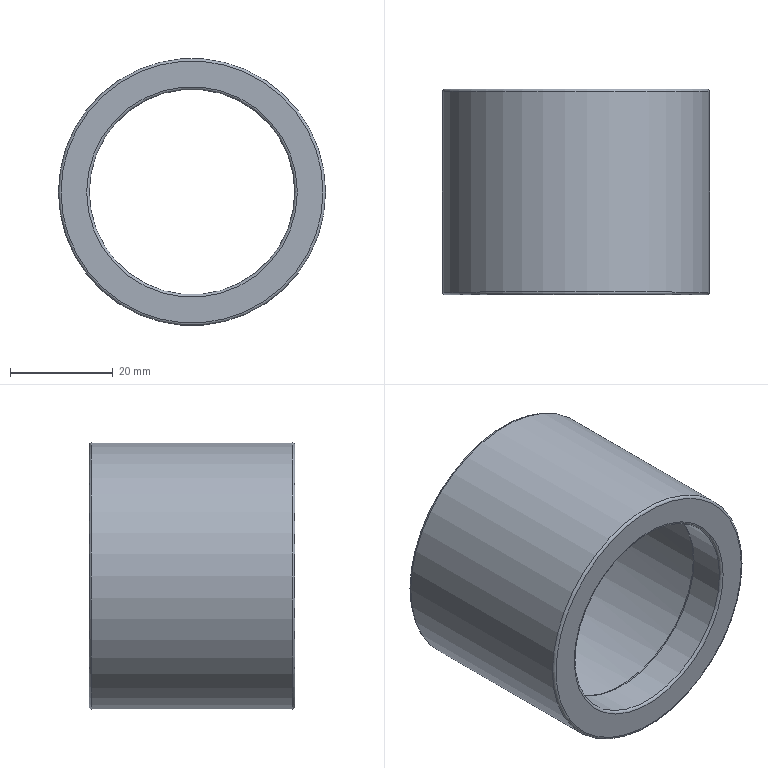Component | NX | 10_THIN_SLEEVE | 1 solid | 16 faces | box 52 x 40 x 52 mm | volume 21385 mm3 | torus 8 | plane 4 | cylinder 4 | commonest cylinder face diameters 40 x2 52 x1 48 x1
STEP:
#1=CARTESIAN_POINT('',(0.,0.,0.));
#2=DIRECTION('',(0.,0.,1.));
#3=DIRECTION('',(1.,0.,0.));
#4=AXIS2_PLACEMENT_3D('',#1,#2,#3);
#5=CARTESIAN_POINT('',(-38.584,152.794,-238.219));
#6=VERTEX_POINT('',#5);
#7=CARTESIAN_POINT('',(-59.084,152.794,-238.219));
#8=DIRECTION('',(0.,-1.,0.));
#9=DIRECTION('',(1.,0.,0.));
#10=AXIS2_PLACEMENT_3D('',#7,#8,#9);
#11=CIRCLE('',#10,20.5);
#12=CARTESIAN_POINT('',(-59.084,152.794,-238.219));
#13=DIRECTION('',(0.,1.,0.));
#14=DIRECTION('',(1.,0.,0.));
#15=AXIS2_PLACEMENT_3D('',#12,#13,#14);
#16=PLANE('',#15);
#17=CARTESIAN_POINT('',(20.5,0.));
#18=CARTESIAN_POINT('',(20.5,-35.507));
#19=CARTESIAN_POINT('',(-10.25,-17.754));
#20=CARTESIAN_POINT('',(-41.,-0.));
#21=CARTESIAN_POINT('',(-10.25,17.754));
#22=CARTESIAN_POINT('',(20.5,35.507));
#23=CARTESIAN_POINT('',(20.5,0.));
#24=(BOUNDED_CURVE()B_SPLINE_CURVE(2,(#17,#18,#19,#20,#21,#22,#23),.UNSPECIFIED.,.T.,.F.)B_SPLINE_CURVE_WITH_KNOTS((1,2,2,2,2,1),(-2.094,0.,2.094,4.189,6.283,8.378),.UNSPECIFIED.)CURVE()GEOMETRIC_REPRESENTATION_ITEM()RATIONAL_B_SPLINE_CURVE((1.,0.5,1.,0.5,1.,0.5,1.))REPRESENTATION_ITEM(''));
#25=(GEOMETRIC_REPRESENTATION_CONTEXT(2)PARAMETRIC_REPRESENTATION_CONTEXT()REPRESENTATION_CONTEXT('',''));
#26=DEFINITIONAL_REPRESENTATION('',(#24),#25);
#27=PCURVE('',#16,#26);
#28=CARTESIAN_POINT('',(-59.084,152.294,-238.219));
#29=DIRECTION('',(0.,1.,0.));
#30=DIRECTION('',(1.,0.,0.));
#31=AXIS2_PLACEMENT_3D('',#28,#29,#30);
#32=TOROIDAL_SURFACE('',#31,20.5,0.5);
#33=CARTESIAN_POINT('',(6.283,7.854));
#34=DIRECTION('',(-1.,0.));
#35=VECTOR('',#34,1.);
#36=LINE('',#33,#35);
#37=(GEOMETRIC_REPRESENTATION_CONTEXT(2)PARAMETRIC_REPRESENTATION_CONTEXT()REPRESENTATION_CONTEXT('',''));
#38=DEFINITIONAL_REPRESENTATION('',(#36),#37);
#39=PCURVE('',#32,#38);
#40=SURFACE_CURVE('',#11,(#27,#39),.PCURVE_S1.);
#41=EDGE_CURVE('',#6,#6,#40,.T.);
#42=ORIENTED_EDGE('',*,*,#41,.T.);
#43=EDGE_LOOP('',(#42));
#44=FACE_BOUND('',#43,.T.);
#45=CARTESIAN_POINT('',(-33.584,152.794,-238.219));
#46=VERTEX_POINT('',#45);
#47=CARTESIAN_POINT('',(-59.084,152.794,-238.219));
#48=DIRECTION('',(0.,1.,0.));
#49=DIRECTION('',(1.,0.,0.));
#50=AXIS2_PLACEMENT_3D('',#47,#48,#49);
#51=CIRCLE('',#50,25.5);
#52=CARTESIAN_POINT('',(0.,0.));
#53=DIRECTION('',(1.,0.));
#54=AXIS2_PLACEMENT_2D('',#52,#53);
#55=CIRCLE('',#54,25.5);
#56=(GEOMETRIC_REPRESENTATION_CONTEXT(2)PARAMETRIC_REPRESENTATION_CONTEXT()REPRESENTATION_CONTEXT('',''));
#57=DEFINITIONAL_REPRESENTATION('',(#55),#56);
#58=PCURVE('',#16,#57);
#59=CARTESIAN_POINT('',(-59.084,152.294,-238.219));
#60=DIRECTION('',(0.,1.,0.));
#61=DIRECTION('',(1.,0.,0.));
#62=AXIS2_PLACEMENT_3D('',#59,#60,#61);
#63=TOROIDAL_SURFACE('',#62,25.5,0.5);
#64=CARTESIAN_POINT('',(0.,7.854));
#65=DIRECTION('',(1.,0.));
#66=VECTOR('',#65,1.);
#67=LINE('',#64,#66);
#68=(GEOMETRIC_REPRESENTATION_CONTEXT(2)PARAMETRIC_REPRESENTATION_CONTEXT()REPRESENTATION_CONTEXT('',''));
#69=DEFINITIONAL_REPRESENTATION('',(#67),#68);
#70=PCURVE('',#63,#69);
#71=SURFACE_CURVE('',#51,(#58,#70),.PCURVE_S1.);
#72=EDGE_CURVE('',#46,#46,#71,.T.);
#73=ORIENTED_EDGE('',*,*,#72,.T.);
#74=EDGE_LOOP('',(#73));
#75=FACE_BOUND('',#74,.T.);
#76=ADVANCED_FACE('',(#44,#75),#16,.T.);
#77=CARTESIAN_POINT('',(-79.584,112.794,-238.219));
#78=VERTEX_POINT('',#77);
#79=CARTESIAN_POINT('',(-59.084,112.794,-238.219));
#80=DIRECTION('',(0.,1.,0.));
#81=DIRECTION('',(-1.,0.,0.));
#82=AXIS2_PLACEMENT_3D('',#79,#80,#81);
#83=CIRCLE('',#82,20.5);
#84=CARTESIAN_POINT('',(-59.084,112.794,-238.219));
#85=DIRECTION('',(0.,-1.,0.));
#86=DIRECTION('',(-1.,0.,0.));
#87=AXIS2_PLACEMENT_3D('',#84,#85,#86);
#88=PLANE('',#87);
#89=CARTESIAN_POINT('',(20.5,0.));
#90=CARTESIAN_POINT('',(20.5,-35.507));
#91=CARTESIAN_POINT('',(-10.25,-17.754));
#92=CARTESIAN_POINT('',(-41.,-0.));
#93=CARTESIAN_POINT('',(-10.25,17.754));
#94=CARTESIAN_POINT('',(20.5,35.507));
#95=CARTESIAN_POINT('',(20.5,0.));
#96=(BOUNDED_CURVE()B_SPLINE_CURVE(2,(#89,#90,#91,#92,#93,#94,#95),.UNSPECIFIED.,.T.,.F.)B_SPLINE_CURVE_WITH_KNOTS((1,2,2,2,2,1),(-2.094,0.,2.094,4.189,6.283,8.378),.UNSPECIFIED.)CURVE()GEOMETRIC_REPRESENTATION_ITEM()RATIONAL_B_SPLINE_CURVE((1.,0.5,1.,0.5,1.,0.5,1.))REPRESENTATION_ITEM(''));
#97=(GEOMETRIC_REPRESENTATION_CONTEXT(2)PARAMETRIC_REPRESENTATION_CONTEXT()REPRESENTATION_CONTEXT('',''));
#98=DEFINITIONAL_REPRESENTATION('',(#96),#97);
#99=PCURVE('',#88,#98);
#100=CARTESIAN_POINT('',(-59.084,113.294,-238.219));
#101=DIRECTION('',(0.,-1.,0.));
#102=DIRECTION('',(-1.,0.,0.));
#103=AXIS2_PLACEMENT_3D('',#100,#101,#102);
#104=TOROIDAL_SURFACE('',#103,20.5,0.5);
#105=CARTESIAN_POINT('',(6.283,7.854));
#106=DIRECTION('',(-1.,0.));
#107=VECTOR('',#106,1.);
#108=LINE('',#105,#107);
#109=(GEOMETRIC_REPRESENTATION_CONTEXT(2)PARAMETRIC_REPRESENTATION_CONTEXT()REPRESENTATION_CONTEXT('',''));
#110=DEFINITIONAL_REPRESENTATION('',(#108),#109);
#111=PCURVE('',#104,#110);
#112=SURFACE_CURVE('',#83,(#99,#111),.PCURVE_S1.);
#113=EDGE_CURVE('',#78,#78,#112,.T.);
#114=ORIENTED_EDGE('',*,*,#113,.T.);
#115=EDGE_LOOP('',(#114));
#116=FACE_BOUND('',#115,.T.);
#117=CARTESIAN_POINT('',(-84.584,112.794,-238.219));
#118=VERTEX_POINT('',#117);
#119=CARTESIAN_POINT('',(-59.084,112.794,-238.219));
#120=DIRECTION('',(0.,-1.,0.));
#121=DIRECTION('',(-1.,0.,0.));
#122=AXIS2_PLACEMENT_3D('',#119,#120,#121);
#123=CIRCLE('',#122,25.5);
#124=CARTESIAN_POINT('',(0.,0.));
#125=DIRECTION('',(1.,0.));
#126=AXIS2_PLACEMENT_2D('',#124,#125);
#127=CIRCLE('',#126,25.5);
#128=(GEOMETRIC_REPRESENTATION_CONTEXT(2)PARAMETRIC_REPRESENTATION_CONTEXT()REPRESENTATION_CONTEXT('',''));
#129=DEFINITIONAL_REPRESENTATION('',(#127),#128);
#130=PCURVE('',#88,#129);
#131=CARTESIAN_POINT('',(-59.084,113.294,-238.219));
#132=DIRECTION('',(0.,-1.,0.));
#133=DIRECTION('',(-1.,0.,0.));
#134=AXIS2_PLACEMENT_3D('',#131,#132,#133);
#135=TOROIDAL_SURFACE('',#134,25.5,0.5);
#136=CARTESIAN_POINT('',(0.,7.854));
#137=DIRECTION('',(1.,0.));
#138=VECTOR('',#137,1.);
#139=LINE('',#136,#138);
#140=(GEOMETRIC_REPRESENTATION_CONTEXT(2)PARAMETRIC_REPRESENTATION_CONTEXT()REPRESENTATION_CONTEXT('',''));
#141=DEFINITIONAL_REPRESENTATION('',(#139),#140);
#142=PCURVE('',#135,#141);
#143=SURFACE_CURVE('',#123,(#130,#142),.PCURVE_S1.);
#144=EDGE_CURVE('',#118,#118,#143,.T.);
#145=ORIENTED_EDGE('',*,*,#144,.T.);
#146=EDGE_LOOP('',(#145));
#147=FACE_BOUND('',#146,.T.);
#148=ADVANCED_FACE('',(#116,#147),#88,.T.);
#149=CARTESIAN_POINT('',(-85.084,113.294,-238.219));
#150=VERTEX_POINT('',#149);
#151=CARTESIAN_POINT('',(-33.084,113.294,-238.219));
#152=VERTEX_POINT('',#151);
#153=CARTESIAN_POINT('',(-59.084,113.294,-238.219));
#154=DIRECTION('',(0.,1.,0.));
#155=DIRECTION('',(-1.,0.,0.));
#156=AXIS2_PLACEMENT_3D('',#153,#154,#155);
#157=CIRCLE('',#156,26.);
#158=CARTESIAN_POINT('',(-59.084,112.794,-238.219));
#159=DIRECTION('',(0.,1.,0.));
#160=DIRECTION('',(1.,0.,0.));
#161=AXIS2_PLACEMENT_3D('',#158,#159,#160);
#162=CYLINDRICAL_SURFACE('',#161,26.);
#163=CARTESIAN_POINT('',(3.142,0.5));
#164=DIRECTION('',(1.,0.));
#165=VECTOR('',#164,1.);
#166=LINE('',#163,#165);
#167=(GEOMETRIC_REPRESENTATION_CONTEXT(2)PARAMETRIC_REPRESENTATION_CONTEXT()REPRESENTATION_CONTEXT('',''));
#168=DEFINITIONAL_REPRESENTATION('',(#166),#167);
#169=PCURVE('',#162,#168);
#170=CARTESIAN_POINT('',(6.283,6.283));
#171=DIRECTION('',(-1.,0.));
#172=VECTOR('',#171,1.);
#173=LINE('',#170,#172);
#174=(GEOMETRIC_REPRESENTATION_CONTEXT(2)PARAMETRIC_REPRESENTATION_CONTEXT()REPRESENTATION_CONTEXT('',''));
#175=DEFINITIONAL_REPRESENTATION('',(#173),#174);
#176=PCURVE('',#135,#175);
#177=SURFACE_CURVE('',#157,(#169,#176),.PCURVE_S1.);
#178=EDGE_CURVE('',#150,#152,#177,.T.);
#179=ORIENTED_EDGE('',*,*,#178,.T.);
#180=CARTESIAN_POINT('',(-33.084,152.294,-238.219));
#181=VERTEX_POINT('',#180);
#182=CARTESIAN_POINT('',(-33.084,113.294,-238.219));
#183=CARTESIAN_POINT('',(-33.084,152.294,-238.219));
#184=B_SPLINE_CURVE_WITH_KNOTS('',1,(#182,#183),.UNSPECIFIED.,.F.,.F.,(2,2),(0.5,39.5),.PIECEWISE_BEZIER_KNOTS.);
#185=CARTESIAN_POINT('',(6.283,0.));
#186=DIRECTION('',(0.,1.));
#187=VECTOR('',#186,1.);
#188=LINE('',#185,#187);
#189=(GEOMETRIC_REPRESENTATION_CONTEXT(2)PARAMETRIC_REPRESENTATION_CONTEXT()REPRESENTATION_CONTEXT('',''));
#190=DEFINITIONAL_REPRESENTATION('',(#188),#189);
#191=PCURVE('',#162,#190);
#192=CARTESIAN_POINT('',(0.,0.));
#193=DIRECTION('',(0.,1.));
#194=VECTOR('',#193,1.);
#195=LINE('',#192,#194);
#196=(GEOMETRIC_REPRESENTATION_CONTEXT(2)PARAMETRIC_REPRESENTATION_CONTEXT()REPRESENTATION_CONTEXT('',''));
#197=DEFINITIONAL_REPRESENTATION('',(#195),#196);
#198=PCURVE('',#162,#197);
#199=SEAM_CURVE('',#184,(#191,#198),.PCURVE_S1.);
#200=EDGE_CURVE('',#152,#181,#199,.T.);
#201=ORIENTED_EDGE('',*,*,#200,.T.);
#202=CARTESIAN_POINT('',(-59.084,152.294,-238.219));
#203=DIRECTION('',(0.,-1.,0.));
#204=DIRECTION('',(1.,0.,0.));
#205=AXIS2_PLACEMENT_3D('',#202,#203,#204);
#206=CIRCLE('',#205,26.);
#207=CARTESIAN_POINT('',(6.283,39.5));
#208=DIRECTION('',(-1.,0.));
#209=VECTOR('',#208,1.);
#210=LINE('',#207,#209);
#211=(GEOMETRIC_REPRESENTATION_CONTEXT(2)PARAMETRIC_REPRESENTATION_CONTEXT()REPRESENTATION_CONTEXT('',''));
#212=DEFINITIONAL_REPRESENTATION('',(#210),#211);
#213=PCURVE('',#162,#212);
#214=CARTESIAN_POINT('',(6.283,6.283));
#215=DIRECTION('',(-1.,0.));
#216=VECTOR('',#215,1.);
#217=LINE('',#214,#216);
#218=(GEOMETRIC_REPRESENTATION_CONTEXT(2)PARAMETRIC_REPRESENTATION_CONTEXT()REPRESENTATION_CONTEXT('',''));
#219=DEFINITIONAL_REPRESENTATION('',(#217),#218);
#220=PCURVE('',#63,#219);
#221=SURFACE_CURVE('',#206,(#213,#220),.PCURVE_S1.);
#222=EDGE_CURVE('',#181,#181,#221,.T.);
#223=ORIENTED_EDGE('',*,*,#222,.T.);
#224=ORIENTED_EDGE('',*,*,#200,.F.);
#225=CARTESIAN_POINT('',(-59.084,113.294,-238.219));
#226=DIRECTION('',(0.,1.,0.));
#227=DIRECTION('',(-1.,0.,0.));
#228=AXIS2_PLACEMENT_3D('',#225,#226,#227);
#229=CIRCLE('',#228,26.);
#230=CARTESIAN_POINT('',(-3.142,0.5));
#231=DIRECTION('',(1.,0.));
#232=VECTOR('',#231,1.);
#233=LINE('',#230,#232);
#234=(GEOMETRIC_REPRESENTATION_CONTEXT(2)PARAMETRIC_REPRESENTATION_CONTEXT()REPRESENTATION_CONTEXT('',''));
#235=DEFINITIONAL_REPRESENTATION('',(#233),#234);
#236=PCURVE('',#162,#235);
#237=CARTESIAN_POINT('',(6.283,6.283));
#238=DIRECTION('',(-1.,0.));
#239=VECTOR('',#238,1.);
#240=LINE('',#237,#239);
#241=(GEOMETRIC_REPRESENTATION_CONTEXT(2)PARAMETRIC_REPRESENTATION_CONTEXT()REPRESENTATION_CONTEXT('',''));
#242=DEFINITIONAL_REPRESENTATION('',(#240),#241);
#243=PCURVE('',#135,#242);
#244=SURFACE_CURVE('',#229,(#236,#243),.PCURVE_S1.);
#245=EDGE_CURVE('',#152,#150,#244,.T.);
#246=ORIENTED_EDGE('',*,*,#245,.T.);
#247=EDGE_LOOP('',(#179,#201,#223,#224,#246));
#248=FACE_BOUND('',#247,.T.);
#249=ADVANCED_FACE('',(#248),#162,.T.);
#250=CARTESIAN_POINT('',(-79.084,120.294,-238.219));
#251=VERTEX_POINT('',#250);
#252=CARTESIAN_POINT('',(-59.084,120.294,-238.219));
#253=DIRECTION('',(0.,1.,0.));
#254=DIRECTION('',(-1.,0.,0.));
#255=AXIS2_PLACEMENT_3D('',#252,#253,#254);
#256=CIRCLE('',#255,20.);
#257=CARTESIAN_POINT('',(-59.084,112.794,-238.219));
#258=DIRECTION('',(0.,1.,0.));
#259=DIRECTION('',(1.,0.,0.));
#260=AXIS2_PLACEMENT_3D('',#257,#258,#259);
#261=CYLINDRICAL_SURFACE('',#260,20.);
#262=CARTESIAN_POINT('',(3.142,7.5));
#263=DIRECTION('',(1.,0.));
#264=VECTOR('',#263,1.);
#265=LINE('',#262,#264);
#266=(GEOMETRIC_REPRESENTATION_CONTEXT(2)PARAMETRIC_REPRESENTATION_CONTEXT()REPRESENTATION_CONTEXT('',''));
#267=DEFINITIONAL_REPRESENTATION('',(#265),#266);
#268=PCURVE('',#261,#267);
#269=CARTESIAN_POINT('',(-59.084,120.294,-238.219));
#270=DIRECTION('',(0.,-1.,0.));
#271=DIRECTION('',(-1.,0.,0.));
#272=AXIS2_PLACEMENT_3D('',#269,#270,#271);
#273=TOROIDAL_SURFACE('',#272,20.5,0.5);
#274=CARTESIAN_POINT('',(6.283,3.142));
#275=DIRECTION('',(-1.,0.));
#276=VECTOR('',#275,1.);
#277=LINE('',#274,#276);
#278=(GEOMETRIC_REPRESENTATION_CONTEXT(2)PARAMETRIC_REPRESENTATION_CONTEXT()REPRESENTATION_CONTEXT('',''));
#279=DEFINITIONAL_REPRESENTATION('',(#277),#278);
#280=PCURVE('',#273,#279);
#281=SURFACE_CURVE('',#256,(#268,#280),.PCURVE_S1.);
#282=EDGE_CURVE('',#251,#251,#281,.T.);
#283=ORIENTED_EDGE('',*,*,#282,.F.);
#284=CARTESIAN_POINT('',(-79.084,113.294,-238.219));
#285=VERTEX_POINT('',#284);
#286=CARTESIAN_POINT('',(-79.084,113.294,-238.219));
#287=CARTESIAN_POINT('',(-79.084,120.294,-238.219));
#288=B_SPLINE_CURVE_WITH_KNOTS('',1,(#286,#287),.UNSPECIFIED.,.F.,.F.,(2,2),(0.5,7.5),.PIECEWISE_BEZIER_KNOTS.);
#289=CARTESIAN_POINT('',(3.142,0.));
#290=DIRECTION('',(0.,1.));
#291=VECTOR('',#290,1.);
#292=LINE('',#289,#291);
#293=(GEOMETRIC_REPRESENTATION_CONTEXT(2)PARAMETRIC_REPRESENTATION_CONTEXT()REPRESENTATION_CONTEXT('',''));
#294=DEFINITIONAL_REPRESENTATION('',(#292),#293);
#295=PCURVE('',#261,#294);
#296=CARTESIAN_POINT('',(9.425,0.));
#297=DIRECTION('',(0.,1.));
#298=VECTOR('',#297,1.);
#299=LINE('',#296,#298);
#300=(GEOMETRIC_REPRESENTATION_CONTEXT(2)PARAMETRIC_REPRESENTATION_CONTEXT()REPRESENTATION_CONTEXT('',''));
#301=DEFINITIONAL_REPRESENTATION('',(#299),#300);
#302=PCURVE('',#261,#301);
#303=SEAM_CURVE('',#288,(#295,#302),.PCURVE_S1.);
#304=EDGE_CURVE('',#285,#251,#303,.T.);
#305=ORIENTED_EDGE('',*,*,#304,.F.);
#306=CARTESIAN_POINT('',(-59.084,113.294,-238.219));
#307=DIRECTION('',(0.,-1.,0.));
#308=DIRECTION('',(-1.,0.,0.));
#309=AXIS2_PLACEMENT_3D('',#306,#307,#308);
#310=CIRCLE('',#309,20.);
#311=CARTESIAN_POINT('',(9.425,0.5));
#312=DIRECTION('',(-1.,0.));
#313=VECTOR('',#312,1.);
#314=LINE('',#311,#313);
#315=(GEOMETRIC_REPRESENTATION_CONTEXT(2)PARAMETRIC_REPRESENTATION_CONTEXT()REPRESENTATION_CONTEXT('',''));
#316=DEFINITIONAL_REPRESENTATION('',(#314),#315);
#317=PCURVE('',#261,#316);
#318=CARTESIAN_POINT('',(0.,9.425));
#319=DIRECTION('',(1.,0.));
#320=VECTOR('',#319,1.);
#321=LINE('',#318,#320);
#322=(GEOMETRIC_REPRESENTATION_CONTEXT(2)PARAMETRIC_REPRESENTATION_CONTEXT()REPRESENTATION_CONTEXT('',''));
#323=DEFINITIONAL_REPRESENTATION('',(#321),#322);
#324=PCURVE('',#104,#323);
#325=SURFACE_CURVE('',#310,(#317,#324),.PCURVE_S1.);
#326=EDGE_CURVE('',#285,#285,#325,.T.);
#327=ORIENTED_EDGE('',*,*,#326,.F.);
#328=ORIENTED_EDGE('',*,*,#304,.T.);
#329=EDGE_LOOP('',(#283,#305,#327,#328));
#330=FACE_BOUND('',#329,.F.);
#331=ADVANCED_FACE('',(#330),#261,.F.);
#332=CARTESIAN_POINT('',(-39.084,145.294,-238.219));
#333=VERTEX_POINT('',#332);
#334=CARTESIAN_POINT('',(-59.084,145.294,-238.219));
#335=DIRECTION('',(0.,-1.,0.));
#336=DIRECTION('',(1.,0.,0.));
#337=AXIS2_PLACEMENT_3D('',#334,#335,#336);
#338=CIRCLE('',#337,20.);
#339=CARTESIAN_POINT('',(-59.084,152.794,-238.219));
#340=DIRECTION('',(0.,-1.,0.));
#341=DIRECTION('',(1.,0.,0.));
#342=AXIS2_PLACEMENT_3D('',#339,#340,#341);
#343=CYLINDRICAL_SURFACE('',#342,20.);
#344=CARTESIAN_POINT('',(0.,7.5));
#345=DIRECTION('',(1.,0.));
#346=VECTOR('',#345,1.);
#347=LINE('',#344,#346);
#348=(GEOMETRIC_REPRESENTATION_CONTEXT(2)PARAMETRIC_REPRESENTATION_CONTEXT()REPRESENTATION_CONTEXT('',''));
#349=DEFINITIONAL_REPRESENTATION('',(#347),#348);
#350=PCURVE('',#343,#349);
#351=CARTESIAN_POINT('',(-59.084,145.294,-238.219));
#352=DIRECTION('',(0.,1.,0.));
#353=DIRECTION('',(1.,0.,0.));
#354=AXIS2_PLACEMENT_3D('',#351,#352,#353);
#355=TOROIDAL_SURFACE('',#354,20.5,0.5);
#356=CARTESIAN_POINT('',(6.283,3.142));
#357=DIRECTION('',(-1.,0.));
#358=VECTOR('',#357,1.);
#359=LINE('',#356,#358);
#360=(GEOMETRIC_REPRESENTATION_CONTEXT(2)PARAMETRIC_REPRESENTATION_CONTEXT()REPRESENTATION_CONTEXT('',''));
#361=DEFINITIONAL_REPRESENTATION('',(#359),#360);
#362=PCURVE('',#355,#361);
#363=SURFACE_CURVE('',#338,(#350,#362),.PCURVE_S1.);
#364=EDGE_CURVE('',#333,#333,#363,.T.);
#365=ORIENTED_EDGE('',*,*,#364,.F.);
#366=CARTESIAN_POINT('',(-39.084,152.294,-238.219));
#367=VERTEX_POINT('',#366);
#368=CARTESIAN_POINT('',(-39.084,152.294,-238.219));
#369=CARTESIAN_POINT('',(-39.084,145.294,-238.219));
#370=B_SPLINE_CURVE_WITH_KNOTS('',1,(#368,#369),.UNSPECIFIED.,.F.,.F.,(2,2),(0.5,7.5),.PIECEWISE_BEZIER_KNOTS.);
#371=CARTESIAN_POINT('',(0.,0.));
#372=DIRECTION('',(0.,1.));
#373=VECTOR('',#372,1.);
#374=LINE('',#371,#373);
#375=(GEOMETRIC_REPRESENTATION_CONTEXT(2)PARAMETRIC_REPRESENTATION_CONTEXT()REPRESENTATION_CONTEXT('',''));
#376=DEFINITIONAL_REPRESENTATION('',(#374),#375);
#377=PCURVE('',#343,#376);
#378=CARTESIAN_POINT('',(6.283,0.));
#379=DIRECTION('',(0.,1.));
#380=VECTOR('',#379,1.);
#381=LINE('',#378,#380);
#382=(GEOMETRIC_REPRESENTATION_CONTEXT(2)PARAMETRIC_REPRESENTATION_CONTEXT()REPRESENTATION_CONTEXT('',''));
#383=DEFINITIONAL_REPRESENTATION('',(#381),#382);
#384=PCURVE('',#343,#383);
#385=SEAM_CURVE('',#370,(#377,#384),.PCURVE_S1.);
#386=EDGE_CURVE('',#367,#333,#385,.T.);
#387=ORIENTED_EDGE('',*,*,#386,.F.);
#388=CARTESIAN_POINT('',(-59.084,152.294,-238.219));
#389=DIRECTION('',(0.,1.,0.));
#390=DIRECTION('',(1.,0.,0.));
#391=AXIS2_PLACEMENT_3D('',#388,#389,#390);
#392=CIRCLE('',#391,20.);
#393=CARTESIAN_POINT('',(6.283,0.5));
#394=DIRECTION('',(-1.,0.));
#395=VECTOR('',#394,1.);
#396=LINE('',#393,#395);
#397=(GEOMETRIC_REPRESENTATION_CONTEXT(2)PARAMETRIC_REPRESENTATION_CONTEXT()REPRESENTATION_CONTEXT('',''));
#398=DEFINITIONAL_REPRESENTATION('',(#396),#397);
#399=PCURVE('',#343,#398);
#400=CARTESIAN_POINT('',(0.,9.425));
#401=DIRECTION('',(1.,0.));
#402=VECTOR('',#401,1.);
#403=LINE('',#400,#402);
#404=(GEOMETRIC_REPRESENTATION_CONTEXT(2)PARAMETRIC_REPRESENTATION_CONTEXT()REPRESENTATION_CONTEXT('',''));
#405=DEFINITIONAL_REPRESENTATION('',(#403),#404);
#406=PCURVE('',#32,#405);
#407=SURFACE_CURVE('',#392,(#399,#406),.PCURVE_S1.);
#408=EDGE_CURVE('',#367,#367,#407,.T.);
#409=ORIENTED_EDGE('',*,*,#408,.F.);
#410=ORIENTED_EDGE('',*,*,#386,.T.);
#411=EDGE_LOOP('',(#365,#387,#409,#410));
#412=FACE_BOUND('',#411,.F.);
#413=ADVANCED_FACE('',(#412),#343,.F.);
#414=CARTESIAN_POINT('',(-82.584,120.794,-238.219));
#415=VERTEX_POINT('',#414);
#416=CARTESIAN_POINT('',(-59.084,120.794,-238.219));
#417=DIRECTION('',(0.,1.,0.));
#418=DIRECTION('',(-1.,0.,0.));
#419=AXIS2_PLACEMENT_3D('',#416,#417,#418);
#420=CIRCLE('',#419,23.5);
#421=CARTESIAN_POINT('',(-59.084,120.794,-238.219));
#422=DIRECTION('',(0.,-1.,0.));
#423=DIRECTION('',(-1.,0.,0.));
#424=AXIS2_PLACEMENT_3D('',#421,#422,#423);
#425=PLANE('',#424);
#426=CARTESIAN_POINT('',(23.5,0.));
#427=CARTESIAN_POINT('',(23.5,-40.703));
#428=CARTESIAN_POINT('',(-11.75,-20.352));
#429=CARTESIAN_POINT('',(-47.,-0.));
#430=CARTESIAN_POINT('',(-11.75,20.352));
#431=CARTESIAN_POINT('',(23.5,40.703));
#432=CARTESIAN_POINT('',(23.5,0.));
#433=(BOUNDED_CURVE()B_SPLINE_CURVE(2,(#426,#427,#428,#429,#430,#431,#432),.UNSPECIFIED.,.T.,.F.)B_SPLINE_CURVE_WITH_KNOTS((1,2,2,2,2,1),(-2.094,0.,2.094,4.189,6.283,8.378),.UNSPECIFIED.)CURVE()GEOMETRIC_REPRESENTATION_ITEM()RATIONAL_B_SPLINE_CURVE((1.,0.5,1.,0.5,1.,0.5,1.))REPRESENTATION_ITEM(''));
#434=(GEOMETRIC_REPRESENTATION_CONTEXT(2)PARAMETRIC_REPRESENTATION_CONTEXT()REPRESENTATION_CONTEXT('',''));
#435=DEFINITIONAL_REPRESENTATION('',(#433),#434);
#436=PCURVE('',#425,#435);
#437=CARTESIAN_POINT('',(-59.084,121.294,-238.219));
#438=DIRECTION('',(0.,-1.,0.));
#439=DIRECTION('',(-1.,0.,0.));
#440=AXIS2_PLACEMENT_3D('',#437,#438,#439);
#441=TOROIDAL_SURFACE('',#440,23.5,0.5);
#442=CARTESIAN_POINT('',(6.283,7.854));
#443=DIRECTION('',(-1.,0.));
#444=VECTOR('',#443,1.);
#445=LINE('',#442,#444);
#446=(GEOMETRIC_REPRESENTATION_CONTEXT(2)PARAMETRIC_REPRESENTATION_CONTEXT()REPRESENTATION_CONTEXT('',''));
#447=DEFINITIONAL_REPRESENTATION('',(#445),#446);
#448=PCURVE('',#441,#447);
#449=SURFACE_CURVE('',#420,(#436,#448),.PCURVE_S1.);
#450=EDGE_CURVE('',#415,#415,#449,.T.);
#451=ORIENTED_EDGE('',*,*,#450,.T.);
#452=EDGE_LOOP('',(#451));
#453=FACE_BOUND('',#452,.T.);
#454=CARTESIAN_POINT('',(-79.584,120.794,-238.219));
#455=VERTEX_POINT('',#454);
#456=CARTESIAN_POINT('',(-59.084,120.794,-238.219));
#457=DIRECTION('',(0.,-1.,0.));
#458=DIRECTION('',(-1.,0.,0.));
#459=AXIS2_PLACEMENT_3D('',#456,#457,#458);
#460=CIRCLE('',#459,20.5);
#461=CARTESIAN_POINT('',(0.,0.));
#462=DIRECTION('',(1.,0.));
#463=AXIS2_PLACEMENT_2D('',#461,#462);
#464=CIRCLE('',#463,20.5);
#465=(GEOMETRIC_REPRESENTATION_CONTEXT(2)PARAMETRIC_REPRESENTATION_CONTEXT()REPRESENTATION_CONTEXT('',''));
#466=DEFINITIONAL_REPRESENTATION('',(#464),#465);
#467=PCURVE('',#425,#466);
#468=CARTESIAN_POINT('',(0.,4.712));
#469=DIRECTION('',(1.,0.));
#470=VECTOR('',#469,1.);
#471=LINE('',#468,#470);
#472=(GEOMETRIC_REPRESENTATION_CONTEXT(2)PARAMETRIC_REPRESENTATION_CONTEXT()REPRESENTATION_CONTEXT('',''));
#473=DEFINITIONAL_REPRESENTATION('',(#471),#472);
#474=PCURVE('',#273,#473);
#475=SURFACE_CURVE('',#460,(#467,#474),.PCURVE_S1.);
#476=EDGE_CURVE('',#455,#455,#475,.T.);
#477=ORIENTED_EDGE('',*,*,#476,.T.);
#478=EDGE_LOOP('',(#477));
#479=FACE_BOUND('',#478,.T.);
#480=ADVANCED_FACE('',(#453,#479),#425,.F.);
#481=CARTESIAN_POINT('',(-35.584,144.794,-238.219));
#482=VERTEX_POINT('',#481);
#483=CARTESIAN_POINT('',(-59.084,144.794,-238.219));
#484=DIRECTION('',(0.,-1.,0.));
#485=DIRECTION('',(1.,0.,0.));
#486=AXIS2_PLACEMENT_3D('',#483,#484,#485);
#487=CIRCLE('',#486,23.5);
#488=CARTESIAN_POINT('',(-59.084,144.794,-238.219));
#489=DIRECTION('',(0.,1.,0.));
#490=DIRECTION('',(1.,0.,0.));
#491=AXIS2_PLACEMENT_3D('',#488,#489,#490);
#492=PLANE('',#491);
#493=CARTESIAN_POINT('',(23.5,0.));
#494=CARTESIAN_POINT('',(23.5,-40.703));
#495=CARTESIAN_POINT('',(-11.75,-20.352));
#496=CARTESIAN_POINT('',(-47.,-0.));
#497=CARTESIAN_POINT('',(-11.75,20.352));
#498=CARTESIAN_POINT('',(23.5,40.703));
#499=CARTESIAN_POINT('',(23.5,0.));
#500=(BOUNDED_CURVE()B_SPLINE_CURVE(2,(#493,#494,#495,#496,#497,#498,#499),.UNSPECIFIED.,.T.,.F.)B_SPLINE_CURVE_WITH_KNOTS((1,2,2,2,2,1),(-2.094,0.,2.094,4.189,6.283,8.378),.UNSPECIFIED.)CURVE()GEOMETRIC_REPRESENTATION_ITEM()RATIONAL_B_SPLINE_CURVE((1.,0.5,1.,0.5,1.,0.5,1.))REPRESENTATION_ITEM(''));
#501=(GEOMETRIC_REPRESENTATION_CONTEXT(2)PARAMETRIC_REPRESENTATION_CONTEXT()REPRESENTATION_CONTEXT('',''));
#502=DEFINITIONAL_REPRESENTATION('',(#500),#501);
#503=PCURVE('',#492,#502);
#504=CARTESIAN_POINT('',(-59.084,144.294,-238.219));
#505=DIRECTION('',(0.,1.,0.));
#506=DIRECTION('',(1.,0.,0.));
#507=AXIS2_PLACEMENT_3D('',#504,#505,#506);
#508=TOROIDAL_SURFACE('',#507,23.5,0.5);
#509=CARTESIAN_POINT('',(6.283,7.854));
#510=DIRECTION('',(-1.,0.));
#511=VECTOR('',#510,1.);
#512=LINE('',#509,#511);
#513=(GEOMETRIC_REPRESENTATION_CONTEXT(2)PARAMETRIC_REPRESENTATION_CONTEXT()REPRESENTATION_CONTEXT('',''));
#514=DEFINITIONAL_REPRESENTATION('',(#512),#513);
#515=PCURVE('',#508,#514);
#516=SURFACE_CURVE('',#487,(#503,#515),.PCURVE_S1.);
#517=EDGE_CURVE('',#482,#482,#516,.T.);
#518=ORIENTED_EDGE('',*,*,#517,.T.);
#519=EDGE_LOOP('',(#518));
#520=FACE_BOUND('',#519,.T.);
#521=CARTESIAN_POINT('',(-38.584,144.794,-238.219));
#522=VERTEX_POINT('',#521);
#523=CARTESIAN_POINT('',(-59.084,144.794,-238.219));
#524=DIRECTION('',(0.,1.,0.));
#525=DIRECTION('',(1.,0.,0.));
#526=AXIS2_PLACEMENT_3D('',#523,#524,#525);
#527=CIRCLE('',#526,20.5);
#528=CARTESIAN_POINT('',(0.,0.));
#529=DIRECTION('',(1.,0.));
#530=AXIS2_PLACEMENT_2D('',#528,#529);
#531=CIRCLE('',#530,20.5);
#532=(GEOMETRIC_REPRESENTATION_CONTEXT(2)PARAMETRIC_REPRESENTATION_CONTEXT()REPRESENTATION_CONTEXT('',''));
#533=DEFINITIONAL_REPRESENTATION('',(#531),#532);
#534=PCURVE('',#492,#533);
#535=CARTESIAN_POINT('',(0.,4.712));
#536=DIRECTION('',(1.,0.));
#537=VECTOR('',#536,1.);
#538=LINE('',#535,#537);
#539=(GEOMETRIC_REPRESENTATION_CONTEXT(2)PARAMETRIC_REPRESENTATION_CONTEXT()REPRESENTATION_CONTEXT('',''));
#540=DEFINITIONAL_REPRESENTATION('',(#538),#539);
#541=PCURVE('',#355,#540);
#542=SURFACE_CURVE('',#527,(#534,#541),.PCURVE_S1.);
#543=EDGE_CURVE('',#522,#522,#542,.T.);
#544=ORIENTED_EDGE('',*,*,#543,.T.);
#545=EDGE_LOOP('',(#544));
#546=FACE_BOUND('',#545,.T.);
#547=ADVANCED_FACE('',(#520,#546),#492,.F.);
#548=CARTESIAN_POINT('',(-35.084,121.294,-238.219));
#549=VERTEX_POINT('',#548);
#550=CARTESIAN_POINT('',(-83.084,121.294,-238.219));
#551=VERTEX_POINT('',#550);
#552=CARTESIAN_POINT('',(-59.084,121.294,-238.219));
#553=DIRECTION('',(0.,-1.,0.));
#554=DIRECTION('',(-1.,0.,0.));
#555=AXIS2_PLACEMENT_3D('',#552,#553,#554);
#556=CIRCLE('',#555,24.);
#557=CARTESIAN_POINT('',(-59.084,120.794,-238.219));
#558=DIRECTION('',(0.,1.,0.));
#559=DIRECTION('',(1.,0.,0.));
#560=AXIS2_PLACEMENT_3D('',#557,#558,#559);
#561=CYLINDRICAL_SURFACE('',#560,24.);
#562=CARTESIAN_POINT('',(9.425,0.5));
#563=DIRECTION('',(-1.,0.));
#564=VECTOR('',#563,1.);
#565=LINE('',#562,#564);
#566=(GEOMETRIC_REPRESENTATION_CONTEXT(2)PARAMETRIC_REPRESENTATION_CONTEXT()REPRESENTATION_CONTEXT('',''));
#567=DEFINITIONAL_REPRESENTATION('',(#565),#566);
#568=PCURVE('',#561,#567);
#569=CARTESIAN_POINT('',(0.,6.283));
#570=DIRECTION('',(1.,0.));
#571=VECTOR('',#570,1.);
#572=LINE('',#569,#571);
#573=(GEOMETRIC_REPRESENTATION_CONTEXT(2)PARAMETRIC_REPRESENTATION_CONTEXT()REPRESENTATION_CONTEXT('',''));
#574=DEFINITIONAL_REPRESENTATION('',(#572),#573);
#575=PCURVE('',#441,#574);
#576=SURFACE_CURVE('',#556,(#568,#575),.PCURVE_S1.);
#577=EDGE_CURVE('',#549,#551,#576,.T.);
#578=ORIENTED_EDGE('',*,*,#577,.F.);
#579=CARTESIAN_POINT('',(-35.084,144.294,-238.219));
#580=VERTEX_POINT('',#579);
#581=CARTESIAN_POINT('',(-35.084,121.294,-238.219));
#582=CARTESIAN_POINT('',(-35.084,144.294,-238.219));
#583=B_SPLINE_CURVE_WITH_KNOTS('',1,(#581,#582),.UNSPECIFIED.,.F.,.F.,(2,2),(0.5,23.5),.PIECEWISE_BEZIER_KNOTS.);
#584=CARTESIAN_POINT('',(6.283,0.));
#585=DIRECTION('',(0.,1.));
#586=VECTOR('',#585,1.);
#587=LINE('',#584,#586);
#588=(GEOMETRIC_REPRESENTATION_CONTEXT(2)PARAMETRIC_REPRESENTATION_CONTEXT()REPRESENTATION_CONTEXT('',''));
#589=DEFINITIONAL_REPRESENTATION('',(#587),#588);
#590=PCURVE('',#561,#589);
#591=CARTESIAN_POINT('',(0.,0.));
#592=DIRECTION('',(0.,1.));
#593=VECTOR('',#592,1.);
#594=LINE('',#591,#593);
#595=(GEOMETRIC_REPRESENTATION_CONTEXT(2)PARAMETRIC_REPRESENTATION_CONTEXT()REPRESENTATION_CONTEXT('',''));
#596=DEFINITIONAL_REPRESENTATION('',(#594),#595);
#597=PCURVE('',#561,#596);
#598=SEAM_CURVE('',#583,(#590,#597),.PCURVE_S1.);
#599=EDGE_CURVE('',#549,#580,#598,.T.);
#600=ORIENTED_EDGE('',*,*,#599,.T.);
#601=CARTESIAN_POINT('',(-59.084,144.294,-238.219));
#602=DIRECTION('',(0.,1.,0.));
#603=DIRECTION('',(1.,0.,0.));
#604=AXIS2_PLACEMENT_3D('',#601,#602,#603);
#605=CIRCLE('',#604,24.);
#606=CARTESIAN_POINT('',(0.,23.5));
#607=DIRECTION('',(1.,0.));
#608=VECTOR('',#607,1.);
#609=LINE('',#606,#608);
#610=(GEOMETRIC_REPRESENTATION_CONTEXT(2)PARAMETRIC_REPRESENTATION_CONTEXT()REPRESENTATION_CONTEXT('',''));
#611=DEFINITIONAL_REPRESENTATION('',(#609),#610);
#612=PCURVE('',#561,#611);
#613=CARTESIAN_POINT('',(0.,6.283));
#614=DIRECTION('',(1.,0.));
#615=VECTOR('',#614,1.);
#616=LINE('',#613,#615);
#617=(GEOMETRIC_REPRESENTATION_CONTEXT(2)PARAMETRIC_REPRESENTATION_CONTEXT()REPRESENTATION_CONTEXT('',''));
#618=DEFINITIONAL_REPRESENTATION('',(#616),#617);
#619=PCURVE('',#508,#618);
#620=SURFACE_CURVE('',#605,(#612,#619),.PCURVE_S1.);
#621=EDGE_CURVE('',#580,#580,#620,.T.);
#622=ORIENTED_EDGE('',*,*,#621,.F.);
#623=ORIENTED_EDGE('',*,*,#599,.F.);
#624=CARTESIAN_POINT('',(-59.084,121.294,-238.219));
#625=DIRECTION('',(0.,-1.,0.));
#626=DIRECTION('',(-1.,0.,0.));
#627=AXIS2_PLACEMENT_3D('',#624,#625,#626);
#628=CIRCLE('',#627,24.);
#629=CARTESIAN_POINT('',(3.142,0.5));
#630=DIRECTION('',(-1.,0.));
#631=VECTOR('',#630,1.);
#632=LINE('',#629,#631);
#633=(GEOMETRIC_REPRESENTATION_CONTEXT(2)PARAMETRIC_REPRESENTATION_CONTEXT()REPRESENTATION_CONTEXT('',''));
#634=DEFINITIONAL_REPRESENTATION('',(#632),#633);
#635=PCURVE('',#561,#634);
#636=CARTESIAN_POINT('',(0.,6.283));
#637=DIRECTION('',(1.,0.));
#638=VECTOR('',#637,1.);
#639=LINE('',#636,#638);
#640=(GEOMETRIC_REPRESENTATION_CONTEXT(2)PARAMETRIC_REPRESENTATION_CONTEXT()REPRESENTATION_CONTEXT('',''));
#641=DEFINITIONAL_REPRESENTATION('',(#639),#640);
#642=PCURVE('',#441,#641);
#643=SURFACE_CURVE('',#628,(#635,#642),.PCURVE_S1.);
#644=EDGE_CURVE('',#551,#549,#643,.T.);
#645=ORIENTED_EDGE('',*,*,#644,.F.);
#646=EDGE_LOOP('',(#578,#600,#622,#623,#645));
#647=FACE_BOUND('',#646,.F.);
#648=ADVANCED_FACE('',(#647),#561,.F.);
#649=ORIENTED_EDGE('',*,*,#450,.T.);
#650=CARTESIAN_POINT('',(-83.084,121.294,-238.219));
#651=CARTESIAN_POINT('',(-83.084,121.16,-238.219));
#652=CARTESIAN_POINT('',(-83.041,121.03,-238.219));
#653=CARTESIAN_POINT('',(-82.96,120.918,-238.219));
#654=CARTESIAN_POINT('',(-82.848,120.836,-238.219));
#655=CARTESIAN_POINT('',(-82.717,120.794,-238.219));
#656=CARTESIAN_POINT('',(-82.584,120.794,-238.219));
#657=(BOUNDED_CURVE()B_SPLINE_CURVE(6,(#650,#651,#652,#653,#654,#655,#656),.UNSPECIFIED.,.F.,.F.)B_SPLINE_CURVE_WITH_KNOTS((7,7),(0.,1.571),.PIECEWISE_BEZIER_KNOTS.)CURVE()GEOMETRIC_REPRESENTATION_ITEM()RATIONAL_B_SPLINE_CURVE((1.031,1.01,0.9979,0.994,0.9979,1.01,1.031))REPRESENTATION_ITEM(''));
#658=CARTESIAN_POINT('',(0.,6.283));
#659=DIRECTION('',(0.,1.));
#660=VECTOR('',#659,1.);
#661=LINE('',#658,#660);
#662=(GEOMETRIC_REPRESENTATION_CONTEXT(2)PARAMETRIC_REPRESENTATION_CONTEXT()REPRESENTATION_CONTEXT('',''));
#663=DEFINITIONAL_REPRESENTATION('',(#661),#662);
#664=PCURVE('',#441,#663);
#665=CARTESIAN_POINT('',(6.283,6.283));
#666=DIRECTION('',(0.,1.));
#667=VECTOR('',#666,1.);
#668=LINE('',#665,#667);
#669=(GEOMETRIC_REPRESENTATION_CONTEXT(2)PARAMETRIC_REPRESENTATION_CONTEXT()REPRESENTATION_CONTEXT('',''));
#670=DEFINITIONAL_REPRESENTATION('',(#668),#669);
#671=PCURVE('',#441,#670);
#672=SEAM_CURVE('',#657,(#664,#671),.PCURVE_S1.);
#673=EDGE_CURVE('',#551,#415,#672,.T.);
#674=ORIENTED_EDGE('',*,*,#673,.F.);
#675=ORIENTED_EDGE('',*,*,#644,.T.);
#676=ORIENTED_EDGE('',*,*,#577,.T.);
#677=ORIENTED_EDGE('',*,*,#673,.T.);
#678=EDGE_LOOP('',(#649,#674,#675,#676,#677));
#679=FACE_BOUND('',#678,.F.);
#680=ADVANCED_FACE('',(#679),#441,.F.);
#681=ORIENTED_EDGE('',*,*,#517,.T.);
#682=CARTESIAN_POINT('',(-35.084,144.294,-238.219));
#683=CARTESIAN_POINT('',(-35.084,144.427,-238.219));
#684=CARTESIAN_POINT('',(-35.126,144.557,-238.219));
#685=CARTESIAN_POINT('',(-35.208,144.67,-238.219));
#686=CARTESIAN_POINT('',(-35.32,144.751,-238.219));
#687=CARTESIAN_POINT('',(-35.45,144.794,-238.219));
#688=CARTESIAN_POINT('',(-35.584,144.794,-238.219));
#689=(BOUNDED_CURVE()B_SPLINE_CURVE(6,(#682,#683,#684,#685,#686,#687,#688),.UNSPECIFIED.,.F.,.F.)B_SPLINE_CURVE_WITH_KNOTS((7,7),(0.,1.571),.PIECEWISE_BEZIER_KNOTS.)CURVE()GEOMETRIC_REPRESENTATION_ITEM()RATIONAL_B_SPLINE_CURVE((1.031,1.01,0.9979,0.994,0.9979,1.01,1.031))REPRESENTATION_ITEM(''));
#690=CARTESIAN_POINT('',(0.,6.283));
#691=DIRECTION('',(0.,1.));
#692=VECTOR('',#691,1.);
#693=LINE('',#690,#692);
#694=(GEOMETRIC_REPRESENTATION_CONTEXT(2)PARAMETRIC_REPRESENTATION_CONTEXT()REPRESENTATION_CONTEXT('',''));
#695=DEFINITIONAL_REPRESENTATION('',(#693),#694);
#696=PCURVE('',#508,#695);
#697=CARTESIAN_POINT('',(6.283,6.283));
#698=DIRECTION('',(0.,1.));
#699=VECTOR('',#698,1.);
#700=LINE('',#697,#699);
#701=(GEOMETRIC_REPRESENTATION_CONTEXT(2)PARAMETRIC_REPRESENTATION_CONTEXT()REPRESENTATION_CONTEXT('',''));
#702=DEFINITIONAL_REPRESENTATION('',(#700),#701);
#703=PCURVE('',#508,#702);
#704=SEAM_CURVE('',#689,(#696,#703),.PCURVE_S1.);
#705=EDGE_CURVE('',#580,#482,#704,.T.);
#706=ORIENTED_EDGE('',*,*,#705,.F.);
#707=ORIENTED_EDGE('',*,*,#621,.T.);
#708=ORIENTED_EDGE('',*,*,#705,.T.);
#709=EDGE_LOOP('',(#681,#706,#707,#708));
#710=FACE_BOUND('',#709,.F.);
#711=ADVANCED_FACE('',(#710),#508,.F.);
#712=ORIENTED_EDGE('',*,*,#543,.F.);
#713=CARTESIAN_POINT('',(-39.084,145.294,-238.219));
#714=CARTESIAN_POINT('',(-39.084,145.16,-238.219));
#715=CARTESIAN_POINT('',(-39.041,145.03,-238.219));
#716=CARTESIAN_POINT('',(-38.96,144.918,-238.219));
#717=CARTESIAN_POINT('',(-38.848,144.836,-238.219));
#718=CARTESIAN_POINT('',(-38.717,144.794,-238.219));
#719=CARTESIAN_POINT('',(-38.584,144.794,-238.219));
#720=(BOUNDED_CURVE()B_SPLINE_CURVE(6,(#713,#714,#715,#716,#717,#718,#719),.UNSPECIFIED.,.F.,.F.)B_SPLINE_CURVE_WITH_KNOTS((7,7),(3.142,4.712),.PIECEWISE_BEZIER_KNOTS.)CURVE()GEOMETRIC_REPRESENTATION_ITEM()RATIONAL_B_SPLINE_CURVE((1.031,1.01,0.9979,0.994,0.9979,1.01,1.031))REPRESENTATION_ITEM(''));
#721=CARTESIAN_POINT('',(0.,0.));
#722=DIRECTION('',(0.,1.));
#723=VECTOR('',#722,1.);
#724=LINE('',#721,#723);
#725=(GEOMETRIC_REPRESENTATION_CONTEXT(2)PARAMETRIC_REPRESENTATION_CONTEXT()REPRESENTATION_CONTEXT('',''));
#726=DEFINITIONAL_REPRESENTATION('',(#724),#725);
#727=PCURVE('',#355,#726);
#728=CARTESIAN_POINT('',(6.283,0.));
#729=DIRECTION('',(0.,1.));
#730=VECTOR('',#729,1.);
#731=LINE('',#728,#730);
#732=(GEOMETRIC_REPRESENTATION_CONTEXT(2)PARAMETRIC_REPRESENTATION_CONTEXT()REPRESENTATION_CONTEXT('',''));
#733=DEFINITIONAL_REPRESENTATION('',(#731),#732);
#734=PCURVE('',#355,#733);
#735=SEAM_CURVE('',#720,(#727,#734),.PCURVE_S1.);
#736=EDGE_CURVE('',#333,#522,#735,.T.);
#737=ORIENTED_EDGE('',*,*,#736,.F.);
#738=ORIENTED_EDGE('',*,*,#364,.F.);
#739=ORIENTED_EDGE('',*,*,#736,.T.);
#740=EDGE_LOOP('',(#712,#737,#738,#739));
#741=FACE_BOUND('',#740,.T.);
#742=ADVANCED_FACE('',(#741),#355,.T.);
#743=ORIENTED_EDGE('',*,*,#476,.F.);
#744=CARTESIAN_POINT('',(-79.084,120.294,-238.219));
#745=CARTESIAN_POINT('',(-79.084,120.427,-238.219));
#746=CARTESIAN_POINT('',(-79.126,120.557,-238.219));
#747=CARTESIAN_POINT('',(-79.208,120.67,-238.219));
#748=CARTESIAN_POINT('',(-79.32,120.751,-238.219));
#749=CARTESIAN_POINT('',(-79.45,120.794,-238.219));
#750=CARTESIAN_POINT('',(-79.584,120.794,-238.219));
#751=(BOUNDED_CURVE()B_SPLINE_CURVE(6,(#744,#745,#746,#747,#748,#749,#750),.UNSPECIFIED.,.F.,.F.)B_SPLINE_CURVE_WITH_KNOTS((7,7),(3.142,4.712),.PIECEWISE_BEZIER_KNOTS.)CURVE()GEOMETRIC_REPRESENTATION_ITEM()RATIONAL_B_SPLINE_CURVE((1.031,1.01,0.9979,0.994,0.9979,1.01,1.031))REPRESENTATION_ITEM(''));
#752=CARTESIAN_POINT('',(0.,0.));
#753=DIRECTION('',(0.,1.));
#754=VECTOR('',#753,1.);
#755=LINE('',#752,#754);
#756=(GEOMETRIC_REPRESENTATION_CONTEXT(2)PARAMETRIC_REPRESENTATION_CONTEXT()REPRESENTATION_CONTEXT('',''));
#757=DEFINITIONAL_REPRESENTATION('',(#755),#756);
#758=PCURVE('',#273,#757);
#759=CARTESIAN_POINT('',(6.283,0.));
#760=DIRECTION('',(0.,1.));
#761=VECTOR('',#760,1.);
#762=LINE('',#759,#761);
#763=(GEOMETRIC_REPRESENTATION_CONTEXT(2)PARAMETRIC_REPRESENTATION_CONTEXT()REPRESENTATION_CONTEXT('',''));
#764=DEFINITIONAL_REPRESENTATION('',(#762),#763);
#765=PCURVE('',#273,#764);
#766=SEAM_CURVE('',#751,(#758,#765),.PCURVE_S1.);
#767=EDGE_CURVE('',#251,#455,#766,.T.);
#768=ORIENTED_EDGE('',*,*,#767,.F.);
#769=ORIENTED_EDGE('',*,*,#282,.F.);
#770=ORIENTED_EDGE('',*,*,#767,.T.);
#771=EDGE_LOOP('',(#743,#768,#769,#770));
#772=FACE_BOUND('',#771,.T.);
#773=ADVANCED_FACE('',(#772),#273,.T.);
#774=ORIENTED_EDGE('',*,*,#408,.F.);
#775=CARTESIAN_POINT('',(-38.584,152.794,-238.219));
#776=CARTESIAN_POINT('',(-38.717,152.794,-238.219));
#777=CARTESIAN_POINT('',(-38.848,152.751,-238.219));
#778=CARTESIAN_POINT('',(-38.96,152.67,-238.219));
#779=CARTESIAN_POINT('',(-39.041,152.557,-238.219));
#780=CARTESIAN_POINT('',(-39.084,152.427,-238.219));
#781=CARTESIAN_POINT('',(-39.084,152.294,-238.219));
#782=(BOUNDED_CURVE()B_SPLINE_CURVE(6,(#775,#776,#777,#778,#779,#780,#781),.UNSPECIFIED.,.F.,.F.)B_SPLINE_CURVE_WITH_KNOTS((7,7),(1.571,3.142),.PIECEWISE_BEZIER_KNOTS.)CURVE()GEOMETRIC_REPRESENTATION_ITEM()RATIONAL_B_SPLINE_CURVE((1.031,1.01,0.9979,0.994,0.9979,1.01,1.031))REPRESENTATION_ITEM(''));
#783=CARTESIAN_POINT('',(0.,6.283));
#784=DIRECTION('',(0.,1.));
#785=VECTOR('',#784,1.);
#786=LINE('',#783,#785);
#787=(GEOMETRIC_REPRESENTATION_CONTEXT(2)PARAMETRIC_REPRESENTATION_CONTEXT()REPRESENTATION_CONTEXT('',''));
#788=DEFINITIONAL_REPRESENTATION('',(#786),#787);
#789=PCURVE('',#32,#788);
#790=CARTESIAN_POINT('',(6.283,6.283));
#791=DIRECTION('',(0.,1.));
#792=VECTOR('',#791,1.);
#793=LINE('',#790,#792);
#794=(GEOMETRIC_REPRESENTATION_CONTEXT(2)PARAMETRIC_REPRESENTATION_CONTEXT()REPRESENTATION_CONTEXT('',''));
#795=DEFINITIONAL_REPRESENTATION('',(#793),#794);
#796=PCURVE('',#32,#795);
#797=SEAM_CURVE('',#782,(#789,#796),.PCURVE_S1.);
#798=EDGE_CURVE('',#6,#367,#797,.T.);
#799=ORIENTED_EDGE('',*,*,#798,.F.);
#800=ORIENTED_EDGE('',*,*,#41,.F.);
#801=ORIENTED_EDGE('',*,*,#798,.T.);
#802=EDGE_LOOP('',(#774,#799,#800,#801));
#803=FACE_BOUND('',#802,.T.);
#804=ADVANCED_FACE('',(#803),#32,.T.);
#805=ORIENTED_EDGE('',*,*,#326,.F.);
#806=CARTESIAN_POINT('',(-79.584,112.794,-238.219));
#807=CARTESIAN_POINT('',(-79.45,112.794,-238.219));
#808=CARTESIAN_POINT('',(-79.32,112.836,-238.219));
#809=CARTESIAN_POINT('',(-79.208,112.918,-238.219));
#810=CARTESIAN_POINT('',(-79.126,113.03,-238.219));
#811=CARTESIAN_POINT('',(-79.084,113.16,-238.219));
#812=CARTESIAN_POINT('',(-79.084,113.294,-238.219));
#813=(BOUNDED_CURVE()B_SPLINE_CURVE(6,(#806,#807,#808,#809,#810,#811,#812),.UNSPECIFIED.,.F.,.F.)B_SPLINE_CURVE_WITH_KNOTS((7,7),(1.571,3.142),.PIECEWISE_BEZIER_KNOTS.)CURVE()GEOMETRIC_REPRESENTATION_ITEM()RATIONAL_B_SPLINE_CURVE((1.031,1.01,0.9979,0.994,0.9979,1.01,1.031))REPRESENTATION_ITEM(''));
#814=CARTESIAN_POINT('',(0.,6.283));
#815=DIRECTION('',(0.,1.));
#816=VECTOR('',#815,1.);
#817=LINE('',#814,#816);
#818=(GEOMETRIC_REPRESENTATION_CONTEXT(2)PARAMETRIC_REPRESENTATION_CONTEXT()REPRESENTATION_CONTEXT('',''));
#819=DEFINITIONAL_REPRESENTATION('',(#817),#818);
#820=PCURVE('',#104,#819);
#821=CARTESIAN_POINT('',(6.283,6.283));
#822=DIRECTION('',(0.,1.));
#823=VECTOR('',#822,1.);
#824=LINE('',#821,#823);
#825=(GEOMETRIC_REPRESENTATION_CONTEXT(2)PARAMETRIC_REPRESENTATION_CONTEXT()REPRESENTATION_CONTEXT('',''));
#826=DEFINITIONAL_REPRESENTATION('',(#824),#825);
#827=PCURVE('',#104,#826);
#828=SEAM_CURVE('',#813,(#820,#827),.PCURVE_S1.);
#829=EDGE_CURVE('',#78,#285,#828,.T.);
#830=ORIENTED_EDGE('',*,*,#829,.F.);
#831=ORIENTED_EDGE('',*,*,#113,.F.);
#832=ORIENTED_EDGE('',*,*,#829,.T.);
#833=EDGE_LOOP('',(#805,#830,#831,#832));
#834=FACE_BOUND('',#833,.T.);
#835=ADVANCED_FACE('',(#834),#104,.T.);
#836=ORIENTED_EDGE('',*,*,#144,.F.);
#837=CARTESIAN_POINT('',(-85.084,113.294,-238.219));
#838=CARTESIAN_POINT('',(-85.084,113.16,-238.219));
#839=CARTESIAN_POINT('',(-85.041,113.03,-238.219));
#840=CARTESIAN_POINT('',(-84.96,112.918,-238.219));
#841=CARTESIAN_POINT('',(-84.848,112.836,-238.219));
#842=CARTESIAN_POINT('',(-84.717,112.794,-238.219));
#843=CARTESIAN_POINT('',(-84.584,112.794,-238.219));
#844=(BOUNDED_CURVE()B_SPLINE_CURVE(6,(#837,#838,#839,#840,#841,#842,#843),.UNSPECIFIED.,.F.,.F.)B_SPLINE_CURVE_WITH_KNOTS((7,7),(0.,1.571),.PIECEWISE_BEZIER_KNOTS.)CURVE()GEOMETRIC_REPRESENTATION_ITEM()RATIONAL_B_SPLINE_CURVE((1.031,1.01,0.9979,0.994,0.9979,1.01,1.031))REPRESENTATION_ITEM(''));
#845=CARTESIAN_POINT('',(0.,6.283));
#846=DIRECTION('',(0.,1.));
#847=VECTOR('',#846,1.);
#848=LINE('',#845,#847);
#849=(GEOMETRIC_REPRESENTATION_CONTEXT(2)PARAMETRIC_REPRESENTATION_CONTEXT()REPRESENTATION_CONTEXT('',''));
#850=DEFINITIONAL_REPRESENTATION('',(#848),#849);
#851=PCURVE('',#135,#850);
#852=CARTESIAN_POINT('',(6.283,6.283));
#853=DIRECTION('',(0.,1.));
#854=VECTOR('',#853,1.);
#855=LINE('',#852,#854);
#856=(GEOMETRIC_REPRESENTATION_CONTEXT(2)PARAMETRIC_REPRESENTATION_CONTEXT()REPRESENTATION_CONTEXT('',''));
#857=DEFINITIONAL_REPRESENTATION('',(#855),#856);
#858=PCURVE('',#135,#857);
#859=SEAM_CURVE('',#844,(#851,#858),.PCURVE_S1.);
#860=EDGE_CURVE('',#150,#118,#859,.T.);
#861=ORIENTED_EDGE('',*,*,#860,.F.);
#862=ORIENTED_EDGE('',*,*,#245,.F.);
#863=ORIENTED_EDGE('',*,*,#178,.F.);
#864=ORIENTED_EDGE('',*,*,#860,.T.);
#865=EDGE_LOOP('',(#836,#861,#862,#863,#864));
#866=FACE_BOUND('',#865,.T.);
#867=ADVANCED_FACE('',(#866),#135,.T.);
#868=ORIENTED_EDGE('',*,*,#72,.F.);
#869=CARTESIAN_POINT('',(-33.084,152.294,-238.219));
#870=CARTESIAN_POINT('',(-33.084,152.427,-238.219));
#871=CARTESIAN_POINT('',(-33.126,152.557,-238.219));
#872=CARTESIAN_POINT('',(-33.208,152.67,-238.219));
#873=CARTESIAN_POINT('',(-33.32,152.751,-238.219));
#874=CARTESIAN_POINT('',(-33.45,152.794,-238.219));
#875=CARTESIAN_POINT('',(-33.584,152.794,-238.219));
#876=(BOUNDED_CURVE()B_SPLINE_CURVE(6,(#869,#870,#871,#872,#873,#874,#875),.UNSPECIFIED.,.F.,.F.)B_SPLINE_CURVE_WITH_KNOTS((7,7),(0.,1.571),.PIECEWISE_BEZIER_KNOTS.)CURVE()GEOMETRIC_REPRESENTATION_ITEM()RATIONAL_B_SPLINE_CURVE((1.031,1.01,0.9979,0.994,0.9979,1.01,1.031))REPRESENTATION_ITEM(''));
#877=CARTESIAN_POINT('',(0.,6.283));
#878=DIRECTION('',(0.,1.));
#879=VECTOR('',#878,1.);
#880=LINE('',#877,#879);
#881=(GEOMETRIC_REPRESENTATION_CONTEXT(2)PARAMETRIC_REPRESENTATION_CONTEXT()REPRESENTATION_CONTEXT('',''));
#882=DEFINITIONAL_REPRESENTATION('',(#880),#881);
#883=PCURVE('',#63,#882);
#884=CARTESIAN_POINT('',(6.283,6.283));
#885=DIRECTION('',(0.,1.));
#886=VECTOR('',#885,1.);
#887=LINE('',#884,#886);
#888=(GEOMETRIC_REPRESENTATION_CONTEXT(2)PARAMETRIC_REPRESENTATION_CONTEXT()REPRESENTATION_CONTEXT('',''));
#889=DEFINITIONAL_REPRESENTATION('',(#887),#888);
#890=PCURVE('',#63,#889);
#891=SEAM_CURVE('',#876,(#883,#890),.PCURVE_S1.);
#892=EDGE_CURVE('',#181,#46,#891,.T.);
#893=ORIENTED_EDGE('',*,*,#892,.F.);
#894=ORIENTED_EDGE('',*,*,#222,.F.);
#895=ORIENTED_EDGE('',*,*,#892,.T.);
#896=EDGE_LOOP('',(#868,#893,#894,#895));
#897=FACE_BOUND('',#896,.T.);
#898=ADVANCED_FACE('',(#897),#63,.T.);
#899=CLOSED_SHELL('',(#76,#148,#249,#331,#413,#480,#547,#648,#680,#711,#742,#773,#804,#835,#867,#898));
#900=MANIFOLD_SOLID_BREP('',#899);
#901=(LENGTH_UNIT()NAMED_UNIT(*)SI_UNIT(.MILLI.,.METRE.));
#902=UNCERTAINTY_MEASURE_WITH_UNIT(LENGTH_MEASURE(0.00001),#901,'','');
#903=(NAMED_UNIT(*)PLANE_ANGLE_UNIT()SI_UNIT($,.RADIAN.));
#904=(NAMED_UNIT(*)SI_UNIT($,.STERADIAN.)SOLID_ANGLE_UNIT());
#905=(GEOMETRIC_REPRESENTATION_CONTEXT(3)GLOBAL_UNCERTAINTY_ASSIGNED_CONTEXT((#902))GLOBAL_UNIT_ASSIGNED_CONTEXT((#901,#903,#904))REPRESENTATION_CONTEXT('',''));
#906=ADVANCED_BREP_SHAPE_REPRESENTATION('',(#4,#900),#905);